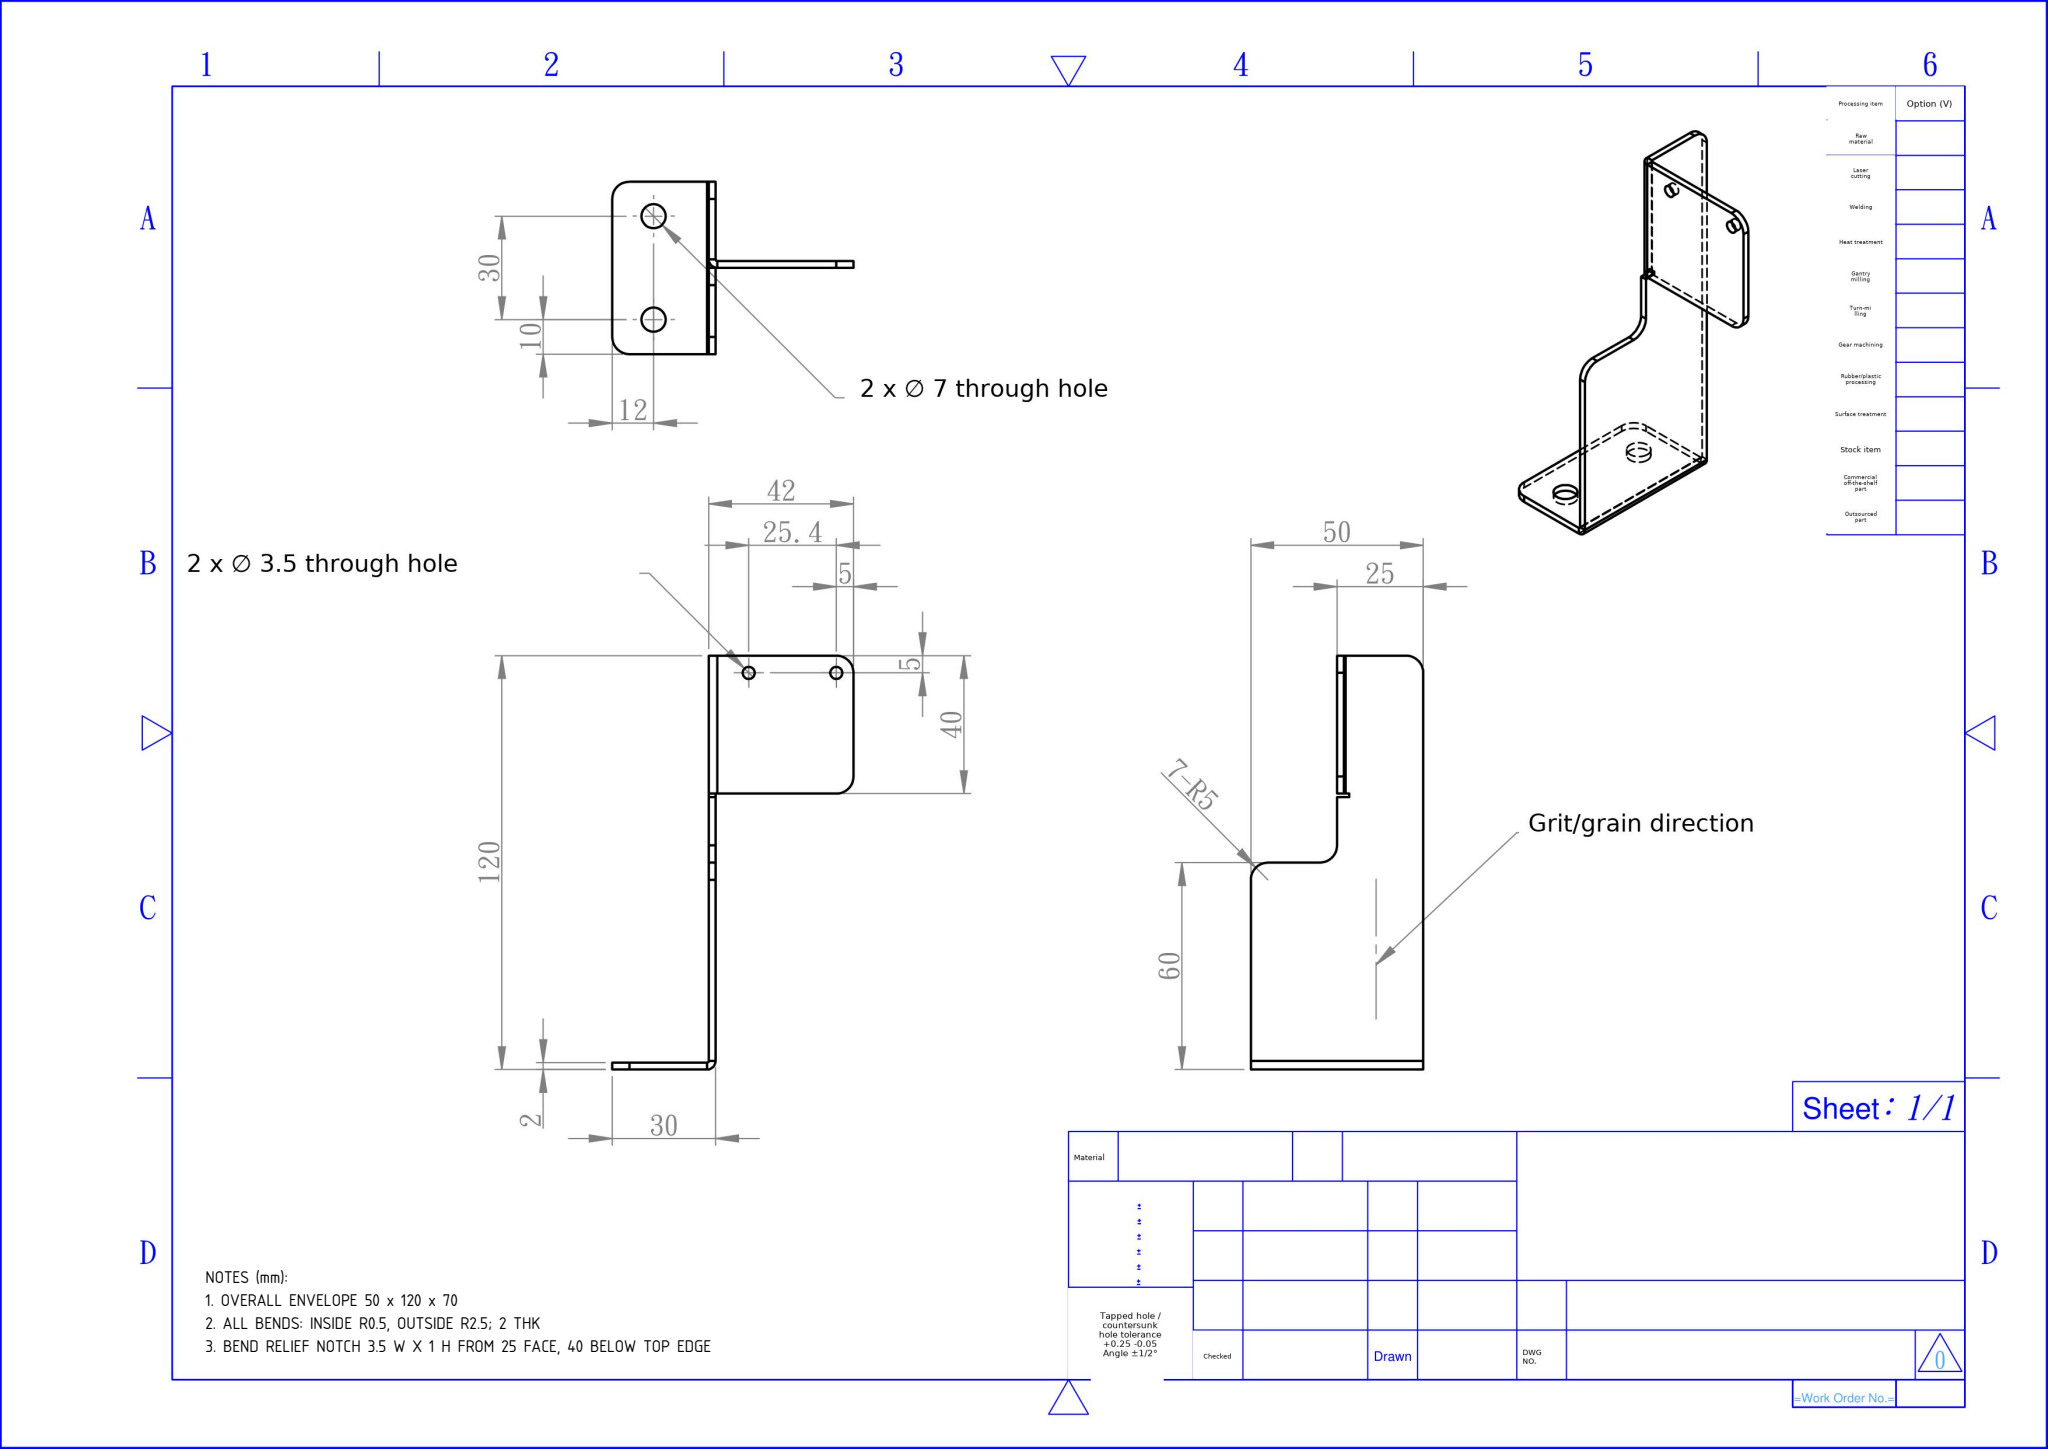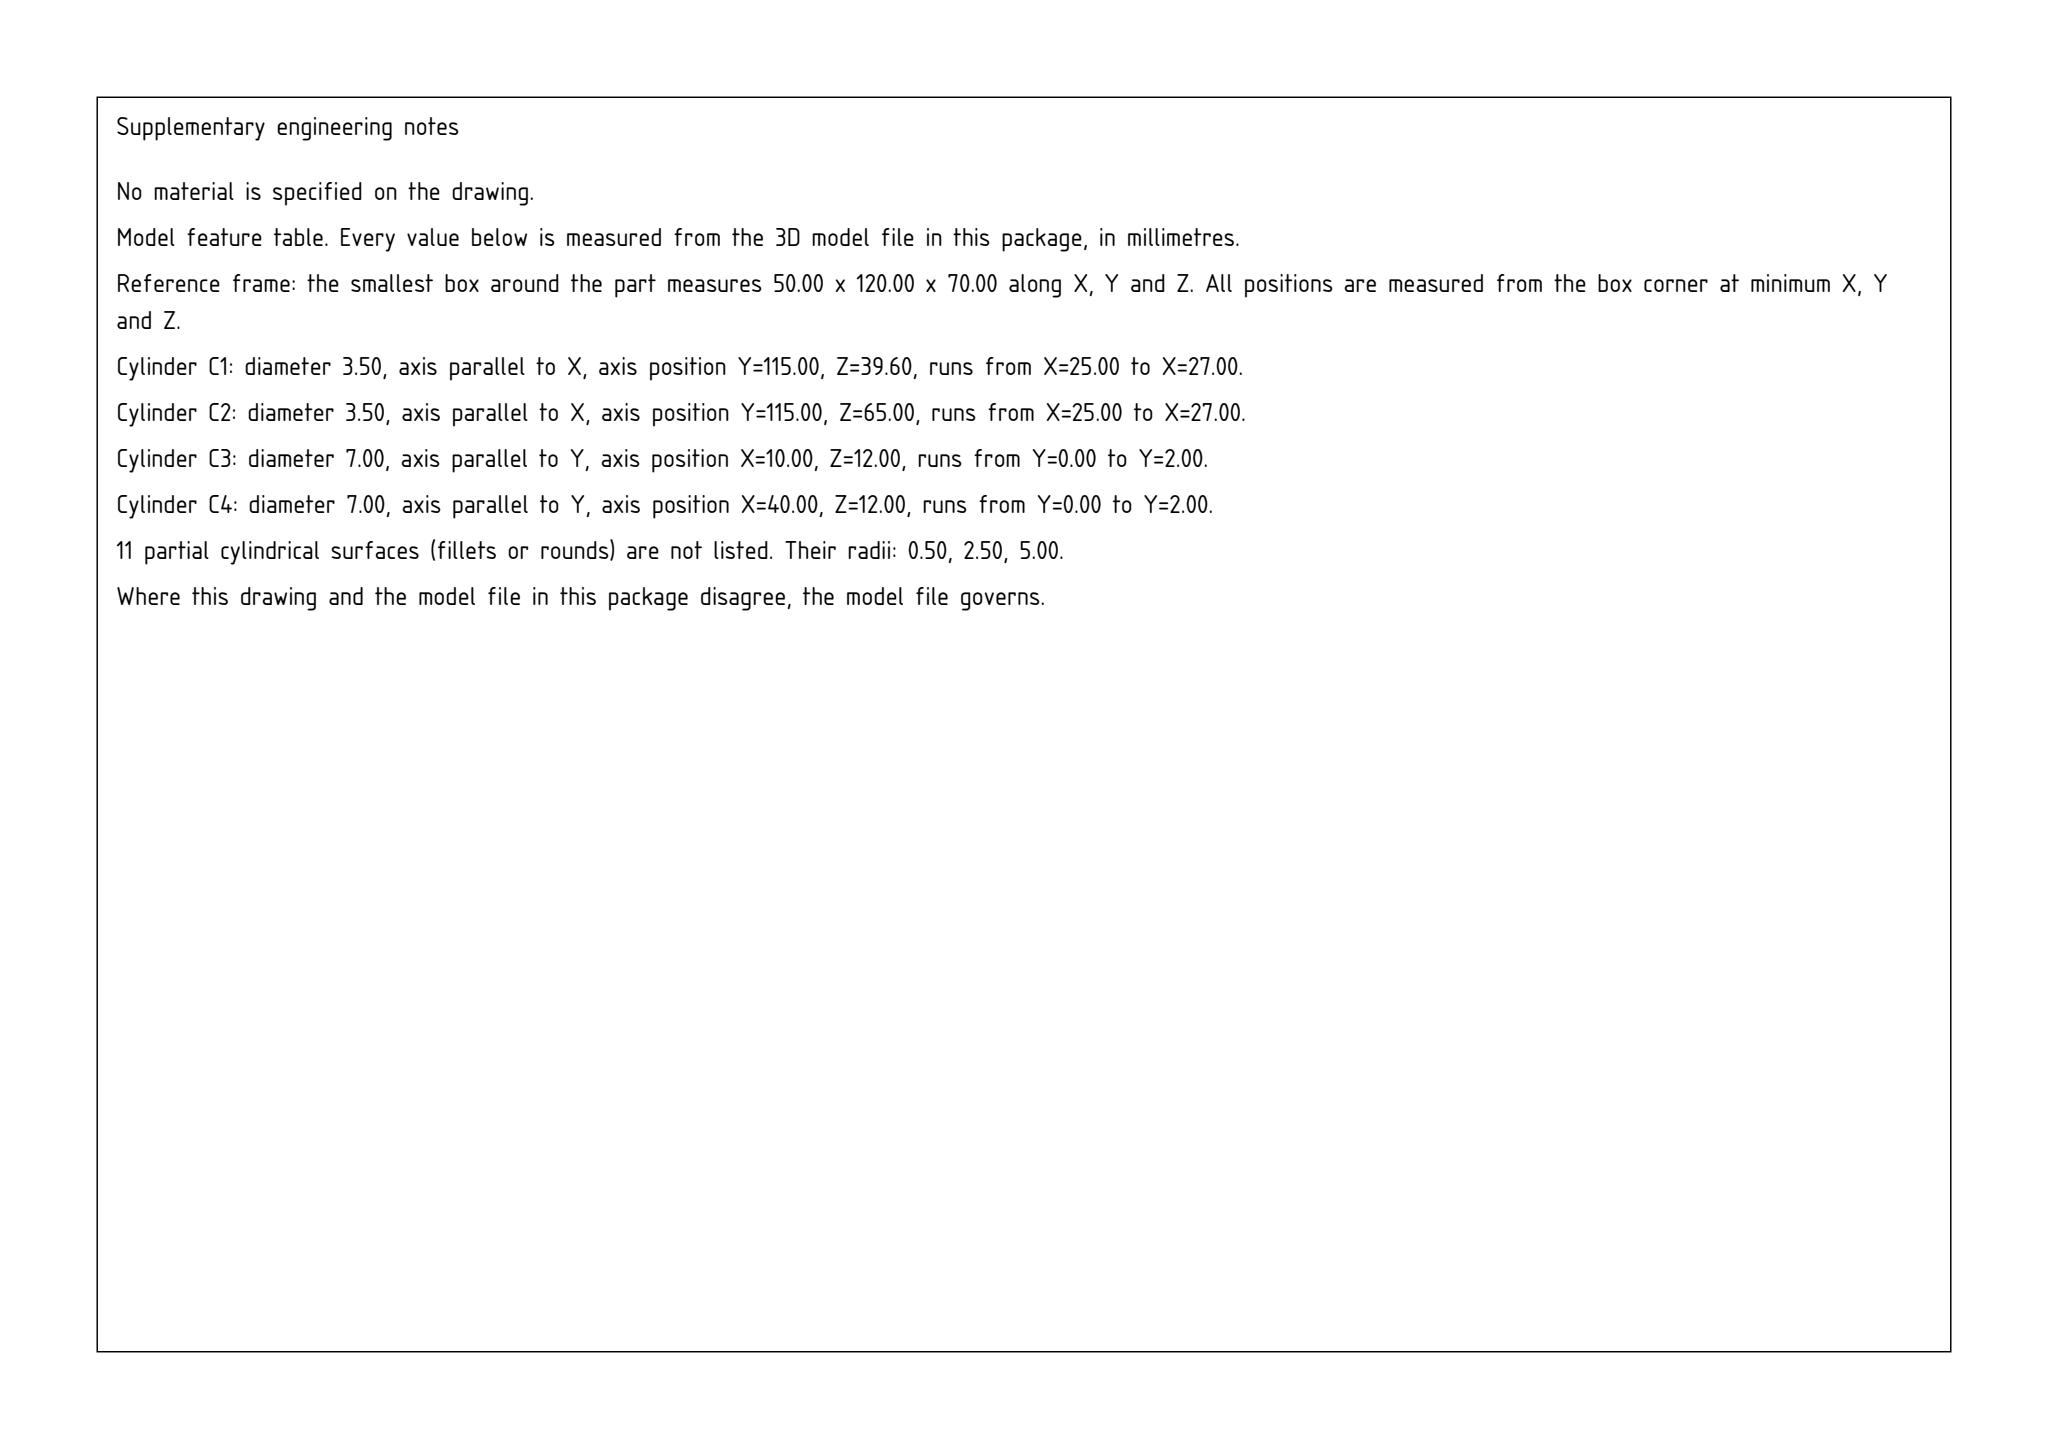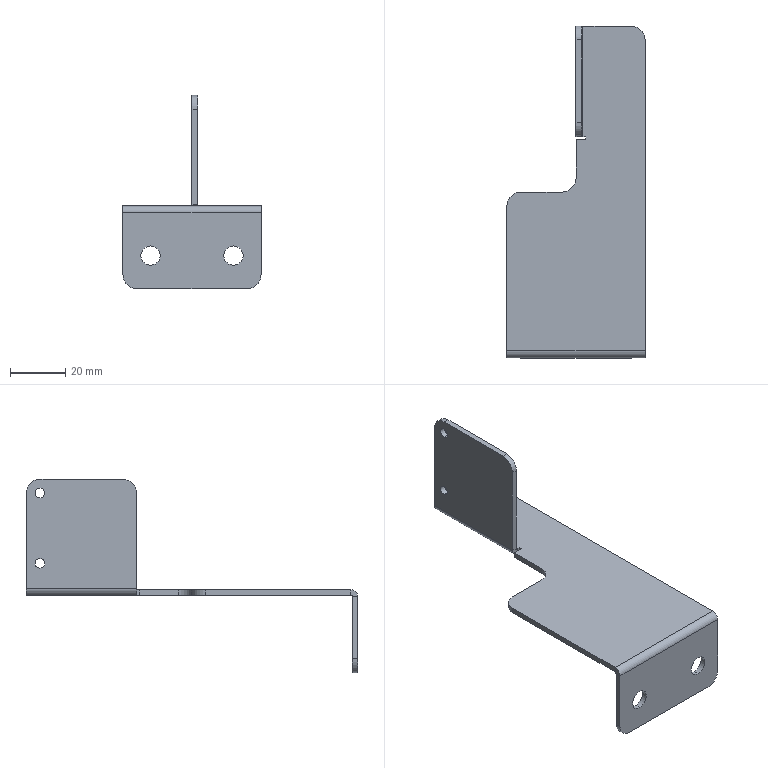Part | SolidWorks | mm | 1 solid | 43 faces | box 50 x 120 x 70 mm | volume 14631 mm3 | plane 24 | cylinder 19 | commonest cylinder face diameters 10 x7 3.5 x4 7 x4 5 x2 1 x2
Drawing notes:
OVERALL ENVELOPE 50 x 120 x 70 | from the solid: bbox_xyz [50.0,120.0,70.0]
ALL BENDS: INSIDE R0.5, OUTSIDE R2.5; 2 THK | from the solid: Bend cyls Ø1.0 (R0.5 inner) & Ø5.0 (R2.5 outer) coaxial at [y2.5,z27.5] and [x27.5,z30.5]; planes y0/y2 = 2 thk
BEND RELIEF NOTCH 3.5 W X 1 H FROM 25 FACE, 40 BELOW TOP EDGE | from the solid: Step faces x=28.5 and y=79 vs x=25 plane and y=80 bend face; top edge y=120 (3.5 wide x 1 high relief at upper bend)